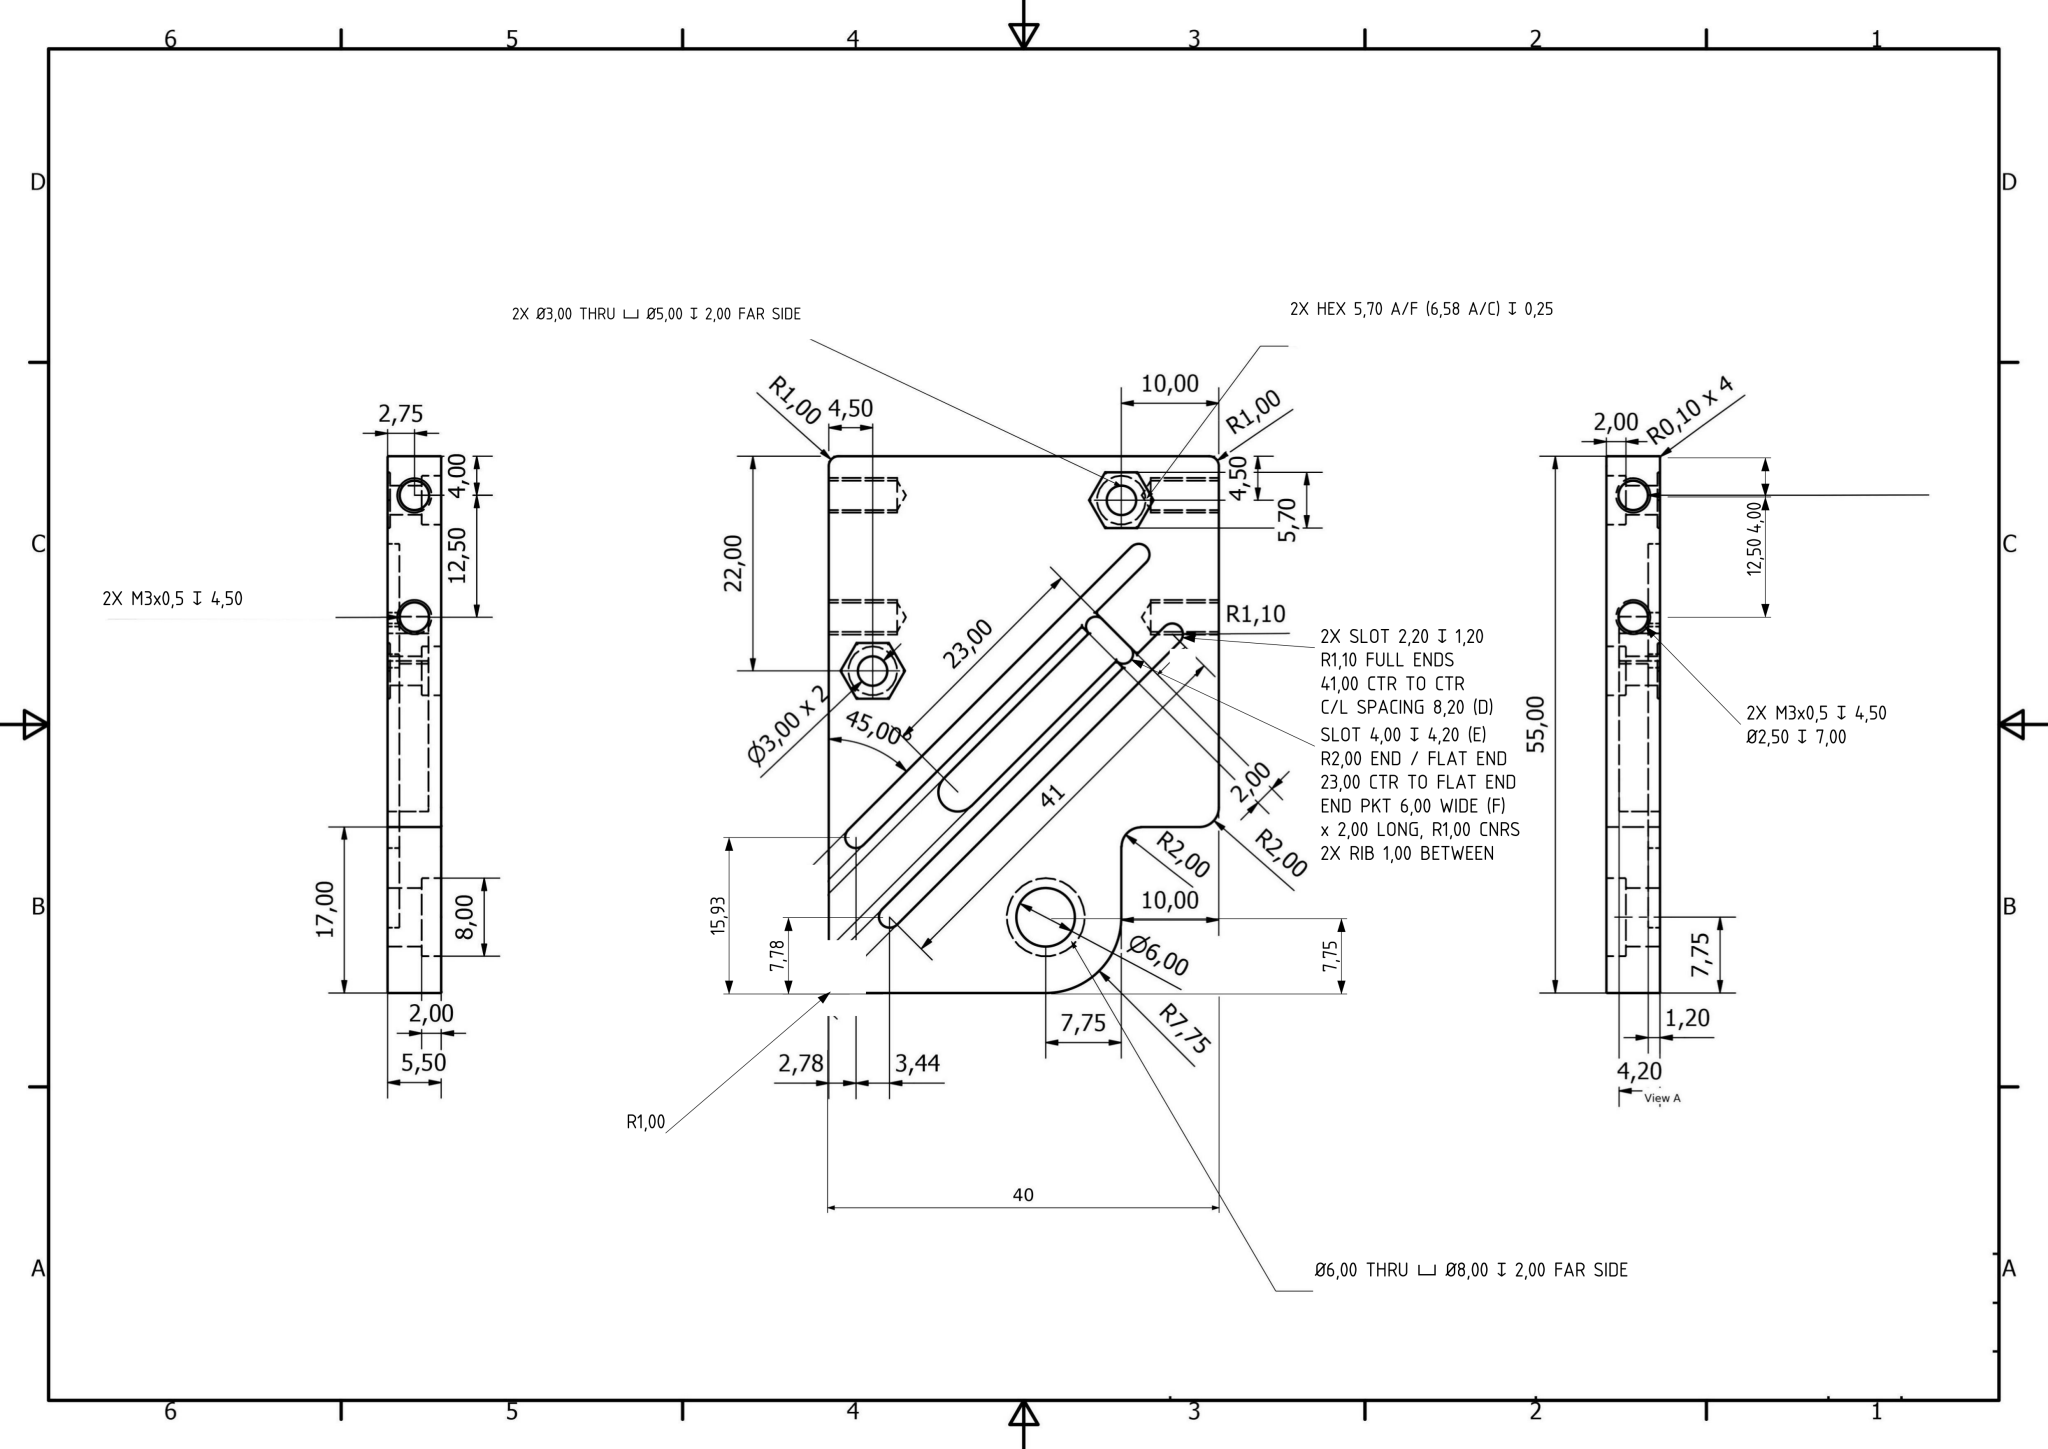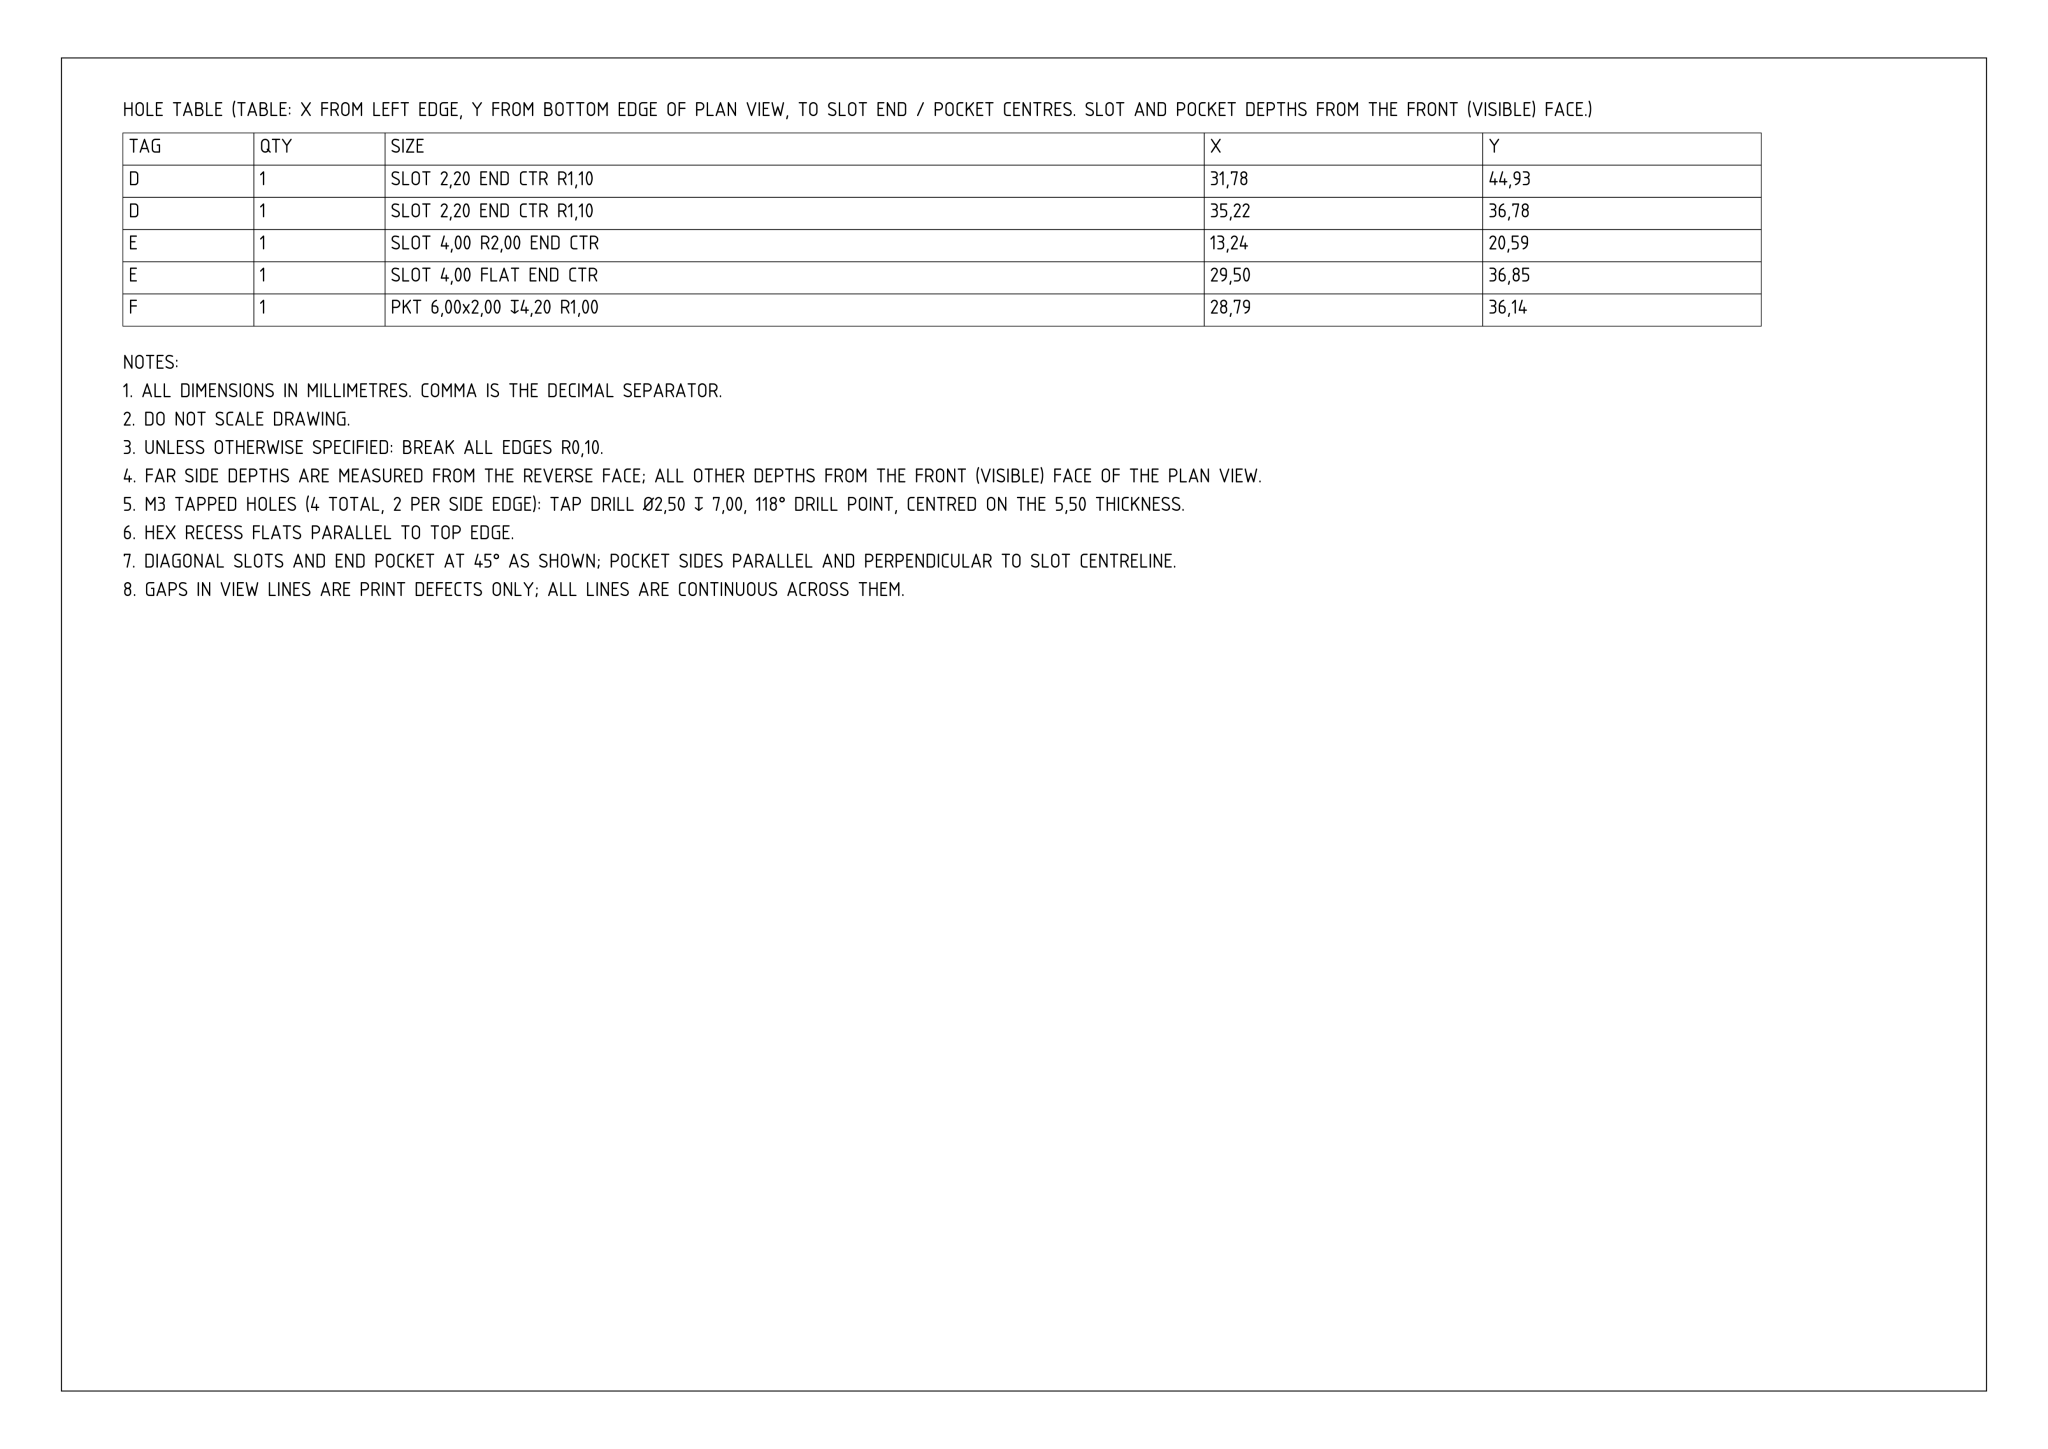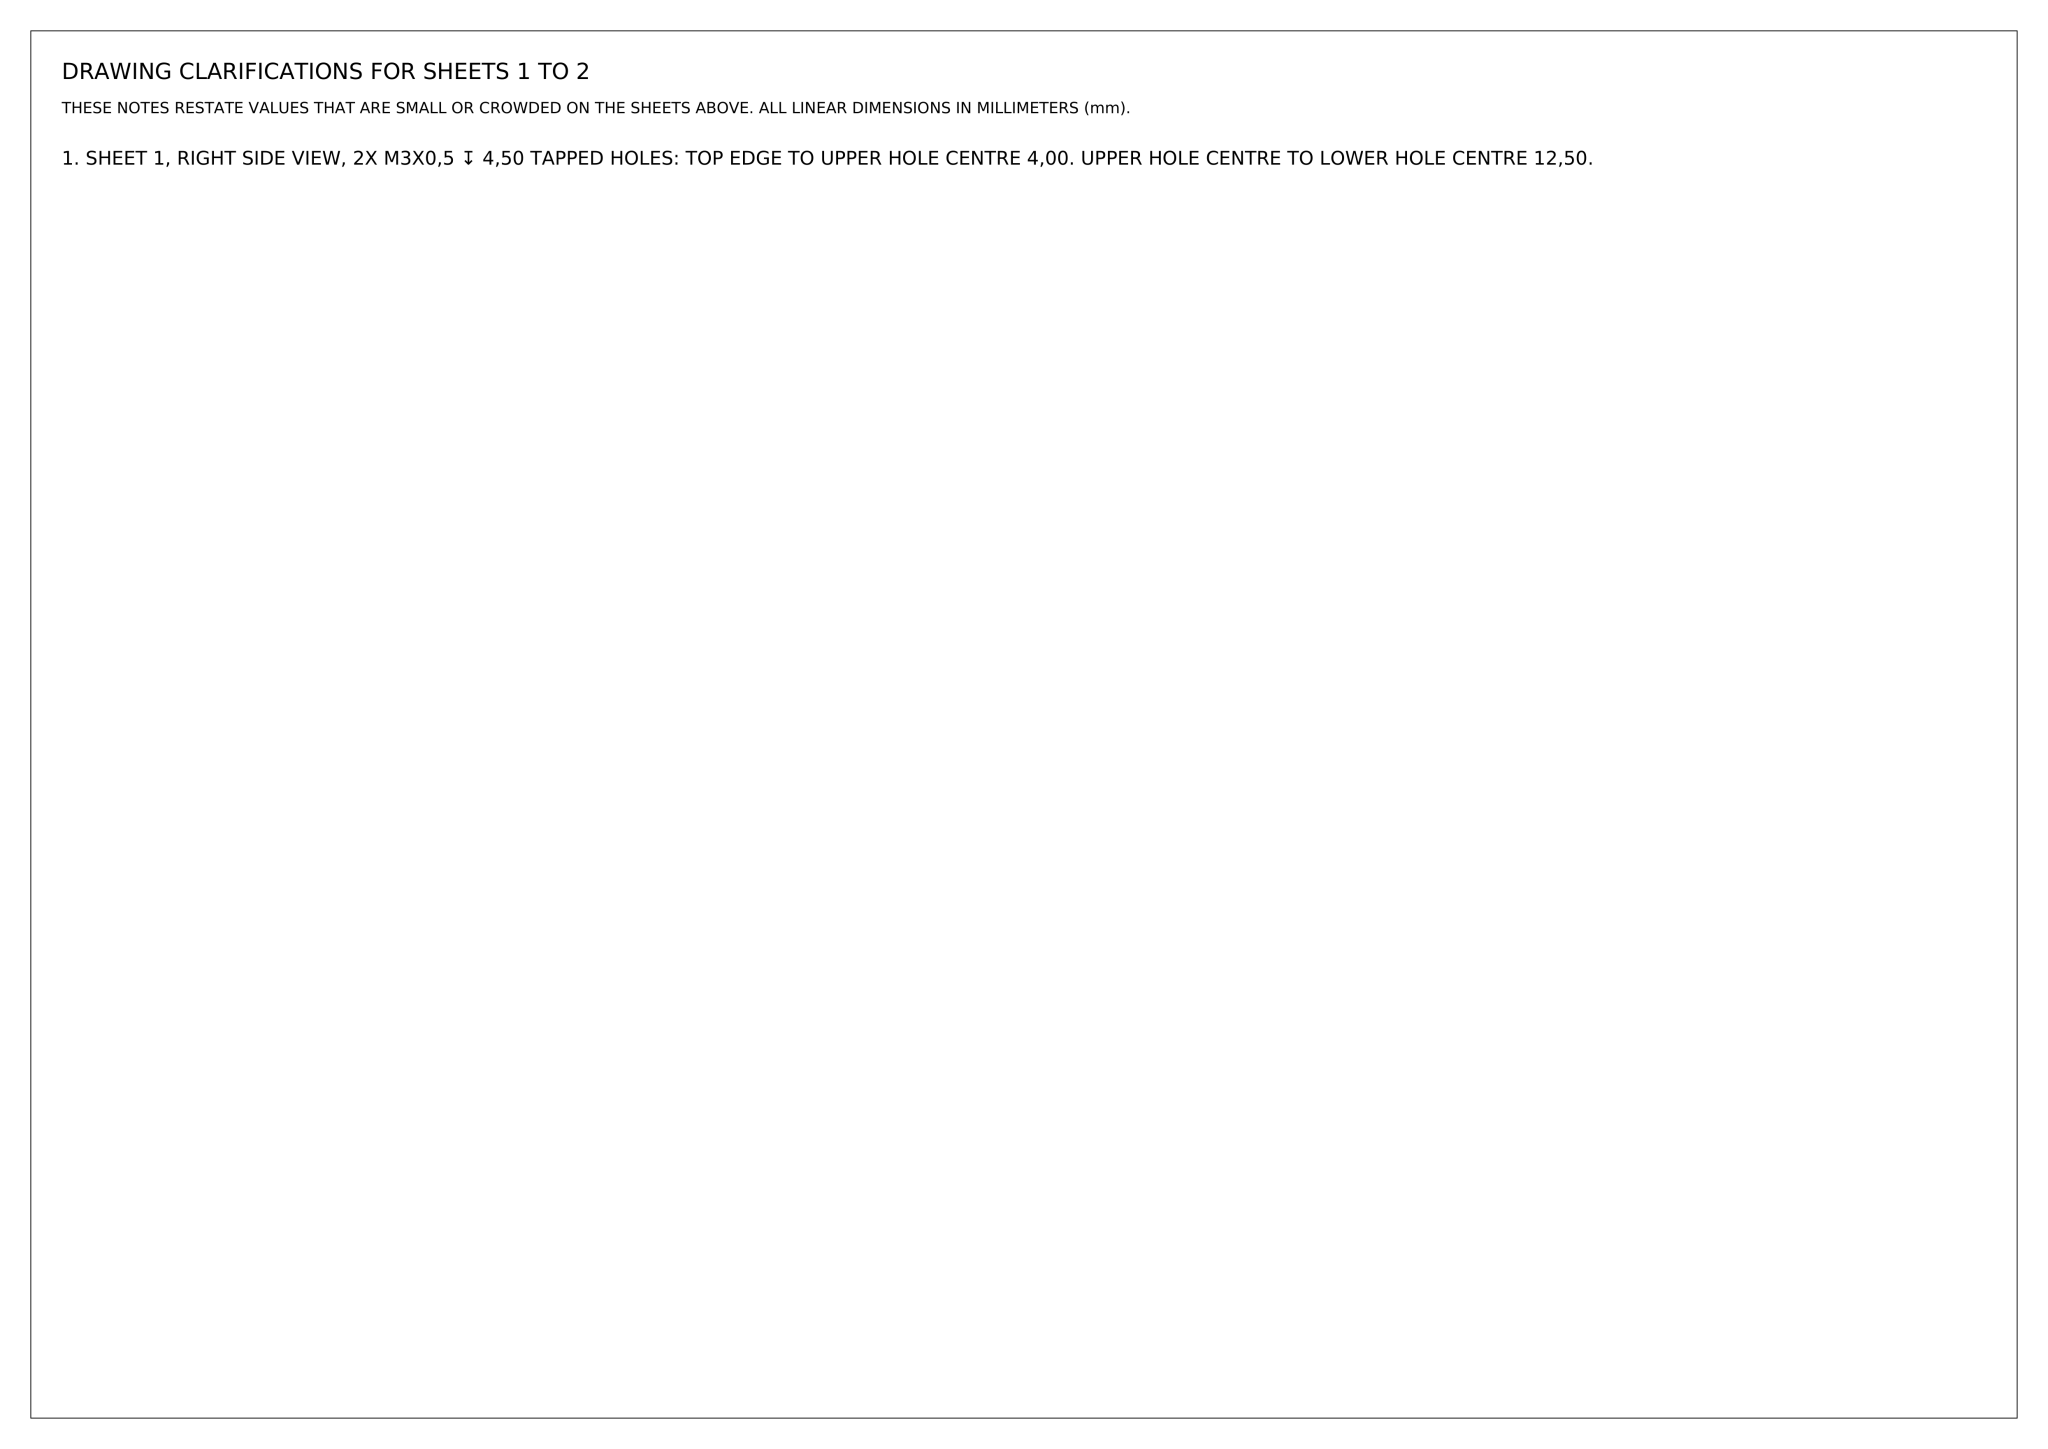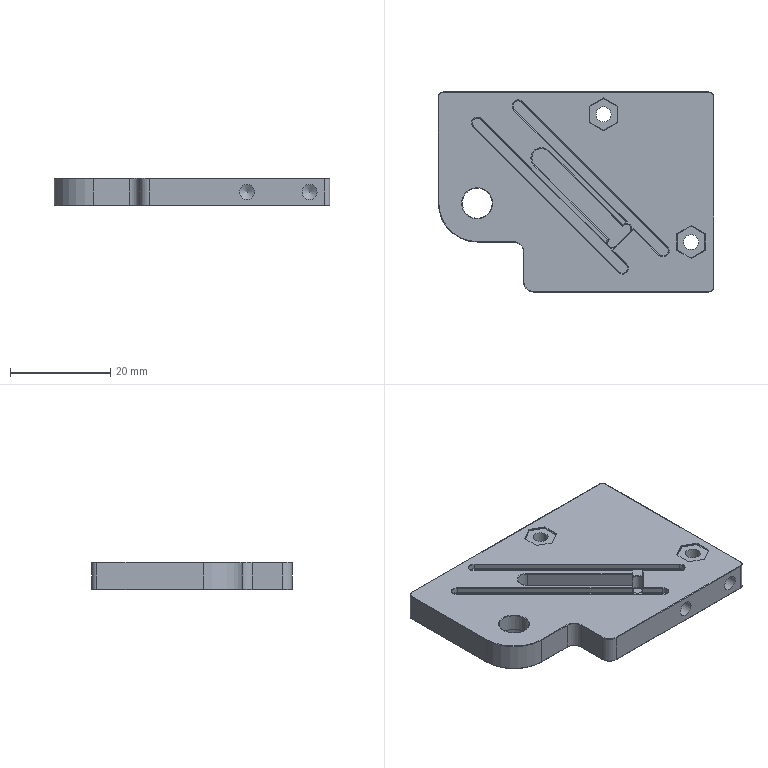Part | NX | mm | 1 solid | 154 faces | box 55 x 40 x 5.5 mm | volume 9893 mm3 | cylinder 71 | plane 39 | torus 36 | cone 4 | spline 4 | commonest cylinder face diameters 0.2 x48 3 x6 2 x5 2.2 x4 4 x3 5 x2 15.5 x1 8 x1